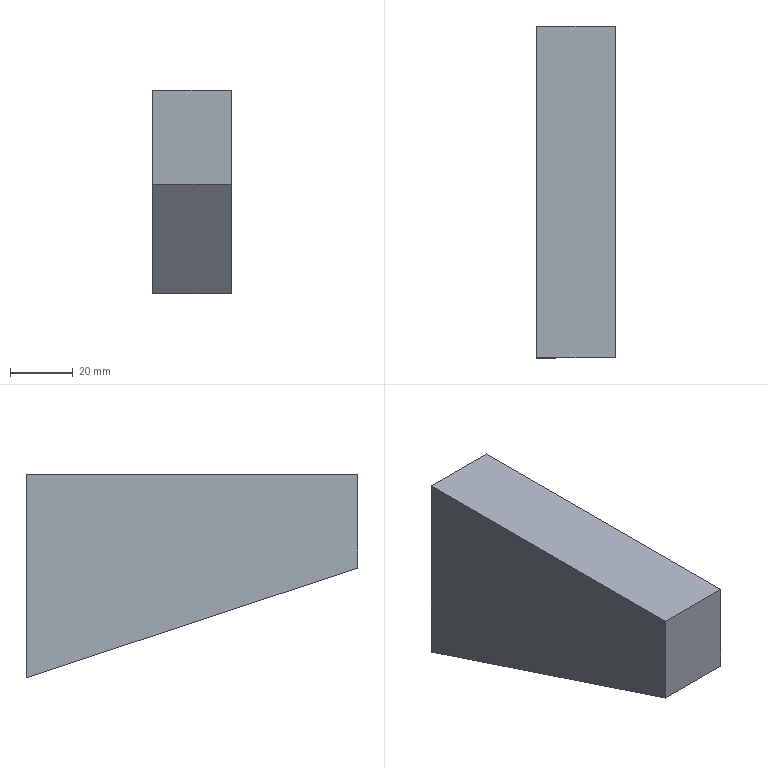Component | SolidWorks | MiddleHousing-1_Stiffener3-1 | 1 solid | 6 faces | box 25 x 106 x 65 mm | volume 125875 mm3 | plane 6
STEP:
#1=CARTESIAN_POINT('',(12.205,1.181,-7.48));
#2=VERTEX_POINT('',#1);
#3=CARTESIAN_POINT('',(12.205,5.354,-8.858));
#4=VERTEX_POINT('',#3);
#5=CARTESIAN_POINT('',(12.205,1.181,-7.48));
#6=DIRECTION('',(0.,0.9496,-0.3135));
#7=VECTOR('',#6,39.37);
#8=LINE('',#5,#7);
#9=EDGE_CURVE('',#2,#4,#8,.T.);
#10=ORIENTED_EDGE('',*,*,#9,.F.);
#11=CARTESIAN_POINT('',(12.205,1.181,-6.299));
#12=VERTEX_POINT('',#11);
#13=CARTESIAN_POINT('',(12.205,1.181,-8.858));
#14=DIRECTION('',(0.,0.,-1.));
#15=VECTOR('',#14,39.37);
#16=LINE('',#13,#15);
#17=EDGE_CURVE('',#12,#2,#16,.T.);
#18=ORIENTED_EDGE('',*,*,#17,.F.);
#19=CARTESIAN_POINT('',(12.205,5.354,-6.299));
#20=VERTEX_POINT('',#19);
#21=CARTESIAN_POINT('',(12.205,5.354,-6.299));
#22=DIRECTION('',(0.,-1.,0.));
#23=VECTOR('',#22,39.37);
#24=LINE('',#21,#23);
#25=EDGE_CURVE('',#20,#12,#24,.T.);
#26=ORIENTED_EDGE('',*,*,#25,.F.);
#27=CARTESIAN_POINT('',(12.205,5.354,-8.858));
#28=DIRECTION('',(0.,0.,1.));
#29=VECTOR('',#28,39.37);
#30=LINE('',#27,#29);
#31=EDGE_CURVE('',#4,#20,#30,.T.);
#32=ORIENTED_EDGE('',*,*,#31,.F.);
#33=EDGE_LOOP('',(#10,#18,#26,#32));
#34=FACE_OUTER_BOUND('',#33,.T.);
#35=CARTESIAN_POINT('',(12.205,5.354,-8.858));
#36=DIRECTION('',(1.,0.,0.));
#37=DIRECTION('',(0.,0.,-1.));
#38=AXIS2_PLACEMENT_3D('',#35,#36,#37);
#39=PLANE('',#38);
#40=ADVANCED_FACE('',(#34),#39,.F.);
#41=CARTESIAN_POINT('',(13.189,5.354,-8.858));
#42=VERTEX_POINT('',#41);
#43=CARTESIAN_POINT('',(13.189,5.354,-6.299));
#44=VERTEX_POINT('',#43);
#45=CARTESIAN_POINT('',(13.189,5.354,-8.858));
#46=DIRECTION('',(0.,0.,1.));
#47=VECTOR('',#46,39.37);
#48=LINE('',#45,#47);
#49=EDGE_CURVE('',#42,#44,#48,.T.);
#50=ORIENTED_EDGE('',*,*,#49,.F.);
#51=CARTESIAN_POINT('',(13.189,5.354,-8.858));
#52=DIRECTION('',(1.,0.,0.));
#53=VECTOR('',#52,39.37);
#54=LINE('',#51,#53);
#55=EDGE_CURVE('',#4,#42,#54,.T.);
#56=ORIENTED_EDGE('',*,*,#55,.F.);
#57=ORIENTED_EDGE('',*,*,#31,.T.);
#58=CARTESIAN_POINT('',(13.189,5.354,-6.299));
#59=DIRECTION('',(-1.,-0.,0.));
#60=VECTOR('',#59,39.37);
#61=LINE('',#58,#60);
#62=EDGE_CURVE('',#44,#20,#61,.T.);
#63=ORIENTED_EDGE('',*,*,#62,.F.);
#64=EDGE_LOOP('',(#50,#56,#57,#63));
#65=FACE_OUTER_BOUND('',#64,.T.);
#66=CARTESIAN_POINT('',(13.189,5.354,-8.858));
#67=DIRECTION('',(0.,-1.,0.));
#68=DIRECTION('',(1.,0.,0.));
#69=AXIS2_PLACEMENT_3D('',#66,#67,#68);
#70=PLANE('',#69);
#71=ADVANCED_FACE('',(#65),#70,.F.);
#72=CARTESIAN_POINT('',(13.189,1.181,-7.48));
#73=VERTEX_POINT('',#72);
#74=CARTESIAN_POINT('',(13.189,5.354,-8.858));
#75=DIRECTION('',(0.,0.9496,-0.3135));
#76=VECTOR('',#75,39.37);
#77=LINE('',#74,#76);
#78=EDGE_CURVE('',#73,#42,#77,.T.);
#79=ORIENTED_EDGE('',*,*,#78,.F.);
#80=CARTESIAN_POINT('',(-2.559,1.181,-7.48));
#81=DIRECTION('',(1.,0.,0.));
#82=VECTOR('',#81,39.37);
#83=LINE('',#80,#82);
#84=EDGE_CURVE('',#2,#73,#83,.T.);
#85=ORIENTED_EDGE('',*,*,#84,.F.);
#86=ORIENTED_EDGE('',*,*,#9,.T.);
#87=ORIENTED_EDGE('',*,*,#55,.T.);
#88=EDGE_LOOP('',(#79,#85,#86,#87));
#89=FACE_OUTER_BOUND('',#88,.T.);
#90=CARTESIAN_POINT('',(-2.559,5.354,-8.858));
#91=DIRECTION('',(0.,0.3135,0.9496));
#92=DIRECTION('',(0.,-0.9496,0.3135));
#93=AXIS2_PLACEMENT_3D('',#90,#91,#92);
#94=PLANE('',#93);
#95=ADVANCED_FACE('',(#89),#94,.F.);
#96=ORIENTED_EDGE('',*,*,#84,.T.);
#97=CARTESIAN_POINT('',(13.189,1.181,-6.299));
#98=VERTEX_POINT('',#97);
#99=CARTESIAN_POINT('',(13.189,1.181,-8.858));
#100=DIRECTION('',(0.,0.,-1.));
#101=VECTOR('',#100,39.37);
#102=LINE('',#99,#101);
#103=EDGE_CURVE('',#98,#73,#102,.T.);
#104=ORIENTED_EDGE('',*,*,#103,.F.);
#105=CARTESIAN_POINT('',(12.205,1.181,-6.299));
#106=DIRECTION('',(1.,0.,0.));
#107=VECTOR('',#106,39.37);
#108=LINE('',#105,#107);
#109=EDGE_CURVE('',#12,#98,#108,.T.);
#110=ORIENTED_EDGE('',*,*,#109,.F.);
#111=ORIENTED_EDGE('',*,*,#17,.T.);
#112=EDGE_LOOP('',(#96,#104,#110,#111));
#113=FACE_OUTER_BOUND('',#112,.T.);
#114=CARTESIAN_POINT('',(12.205,1.181,-8.858));
#115=DIRECTION('',(0.,1.,0.));
#116=DIRECTION('',(0.,0.,1.));
#117=AXIS2_PLACEMENT_3D('',#114,#115,#116);
#118=PLANE('',#117);
#119=ADVANCED_FACE('',(#113),#118,.F.);
#120=ORIENTED_EDGE('',*,*,#25,.T.);
#121=ORIENTED_EDGE('',*,*,#109,.T.);
#122=CARTESIAN_POINT('',(13.189,0.9843,-6.299));
#123=DIRECTION('',(0.,1.,0.));
#124=VECTOR('',#123,39.37);
#125=LINE('',#122,#124);
#126=EDGE_CURVE('',#98,#44,#125,.T.);
#127=ORIENTED_EDGE('',*,*,#126,.T.);
#128=ORIENTED_EDGE('',*,*,#62,.T.);
#129=EDGE_LOOP('',(#120,#121,#127,#128));
#130=FACE_OUTER_BOUND('',#129,.T.);
#131=CARTESIAN_POINT('',(8.268,0.9843,-6.299));
#132=DIRECTION('',(0.,0.,1.));
#133=DIRECTION('',(1.,0.,0.));
#134=AXIS2_PLACEMENT_3D('',#131,#132,#133);
#135=PLANE('',#134);
#136=ADVANCED_FACE('',(#130),#135,.T.);
#137=ORIENTED_EDGE('',*,*,#78,.T.);
#138=ORIENTED_EDGE('',*,*,#49,.T.);
#139=ORIENTED_EDGE('',*,*,#126,.F.);
#140=ORIENTED_EDGE('',*,*,#103,.T.);
#141=EDGE_LOOP('',(#137,#138,#139,#140));
#142=FACE_OUTER_BOUND('',#141,.T.);
#143=CARTESIAN_POINT('',(13.189,1.181,-8.858));
#144=DIRECTION('',(-1.,-0.,0.));
#145=DIRECTION('',(0.,-1.,0.));
#146=AXIS2_PLACEMENT_3D('',#143,#144,#145);
#147=PLANE('',#146);
#148=ADVANCED_FACE('',(#142),#147,.F.);
#149=CLOSED_SHELL('',(#40,#71,#95,#119,#136,#148));
#150=MANIFOLD_SOLID_BREP('',#149);
#151=CARTESIAN_POINT('',(0.,0.,0.));
#152=DIRECTION('',(0.,0.,1.));
#153=DIRECTION('',(1.,0.,0.));
#154=AXIS2_PLACEMENT_3D('',#151,#152,#153);
#155=(LENGTH_UNIT()NAMED_UNIT(*)SI_UNIT($,.METRE.));
#156=LENGTH_MEASURE_WITH_UNIT(LENGTH_MEASURE(0.0254),#155);
#157=DIMENSIONAL_EXPONENTS(1.,0.,0.,0.,0.,0.,0.);
#158=(CONVERSION_BASED_UNIT('',#156)LENGTH_UNIT()NAMED_UNIT(#157));
#159=UNCERTAINTY_MEASURE_WITH_UNIT(LENGTH_MEASURE(0.00001),#158,'','');
#160=(NAMED_UNIT(*)PLANE_ANGLE_UNIT()SI_UNIT($,.RADIAN.));
#161=(NAMED_UNIT(*)SI_UNIT($,.STERADIAN.)SOLID_ANGLE_UNIT());
#162=(GEOMETRIC_REPRESENTATION_CONTEXT(3)GLOBAL_UNCERTAINTY_ASSIGNED_CONTEXT((#159))GLOBAL_UNIT_ASSIGNED_CONTEXT((#158,#160,#161))REPRESENTATION_CONTEXT('',''));
#163=ADVANCED_BREP_SHAPE_REPRESENTATION('',(#150,#154),#162);
#164=COLOUR_RGB('',0.7922,0.8196,0.9333);
#165=FILL_AREA_STYLE_COLOUR('',#164);
#166=FILL_AREA_STYLE('',(#165));
#167=SURFACE_STYLE_FILL_AREA(#166);
#168=SURFACE_SIDE_STYLE('',(#167));
#169=SURFACE_STYLE_USAGE(.BOTH.,#168);
#170=PRESENTATION_STYLE_ASSIGNMENT((#169));
#171=STYLED_ITEM('',(#170),#150);
#172=PRESENTATION_LAYER_ASSIGNMENT('','',(#171));
#173=(LENGTH_UNIT()NAMED_UNIT(*)SI_UNIT($,.METRE.));
#174=LENGTH_MEASURE_WITH_UNIT(LENGTH_MEASURE(0.0254),#173);
#175=DIMENSIONAL_EXPONENTS(1.,0.,0.,0.,0.,0.,0.);
#176=(CONVERSION_BASED_UNIT('',#174)LENGTH_UNIT()NAMED_UNIT(#175));
#177=UNCERTAINTY_MEASURE_WITH_UNIT(LENGTH_MEASURE(0.00001),#176,'','');
#178=(NAMED_UNIT(*)PLANE_ANGLE_UNIT()SI_UNIT($,.RADIAN.));
#179=(NAMED_UNIT(*)SI_UNIT($,.STERADIAN.)SOLID_ANGLE_UNIT());
#180=(GEOMETRIC_REPRESENTATION_CONTEXT(3)GLOBAL_UNCERTAINTY_ASSIGNED_CONTEXT((#177))GLOBAL_UNIT_ASSIGNED_CONTEXT((#176,#178,#179))REPRESENTATION_CONTEXT('',''));
#181=MECHANICAL_DESIGN_GEOMETRIC_PRESENTATION_REPRESENTATION('',(#171),#180);